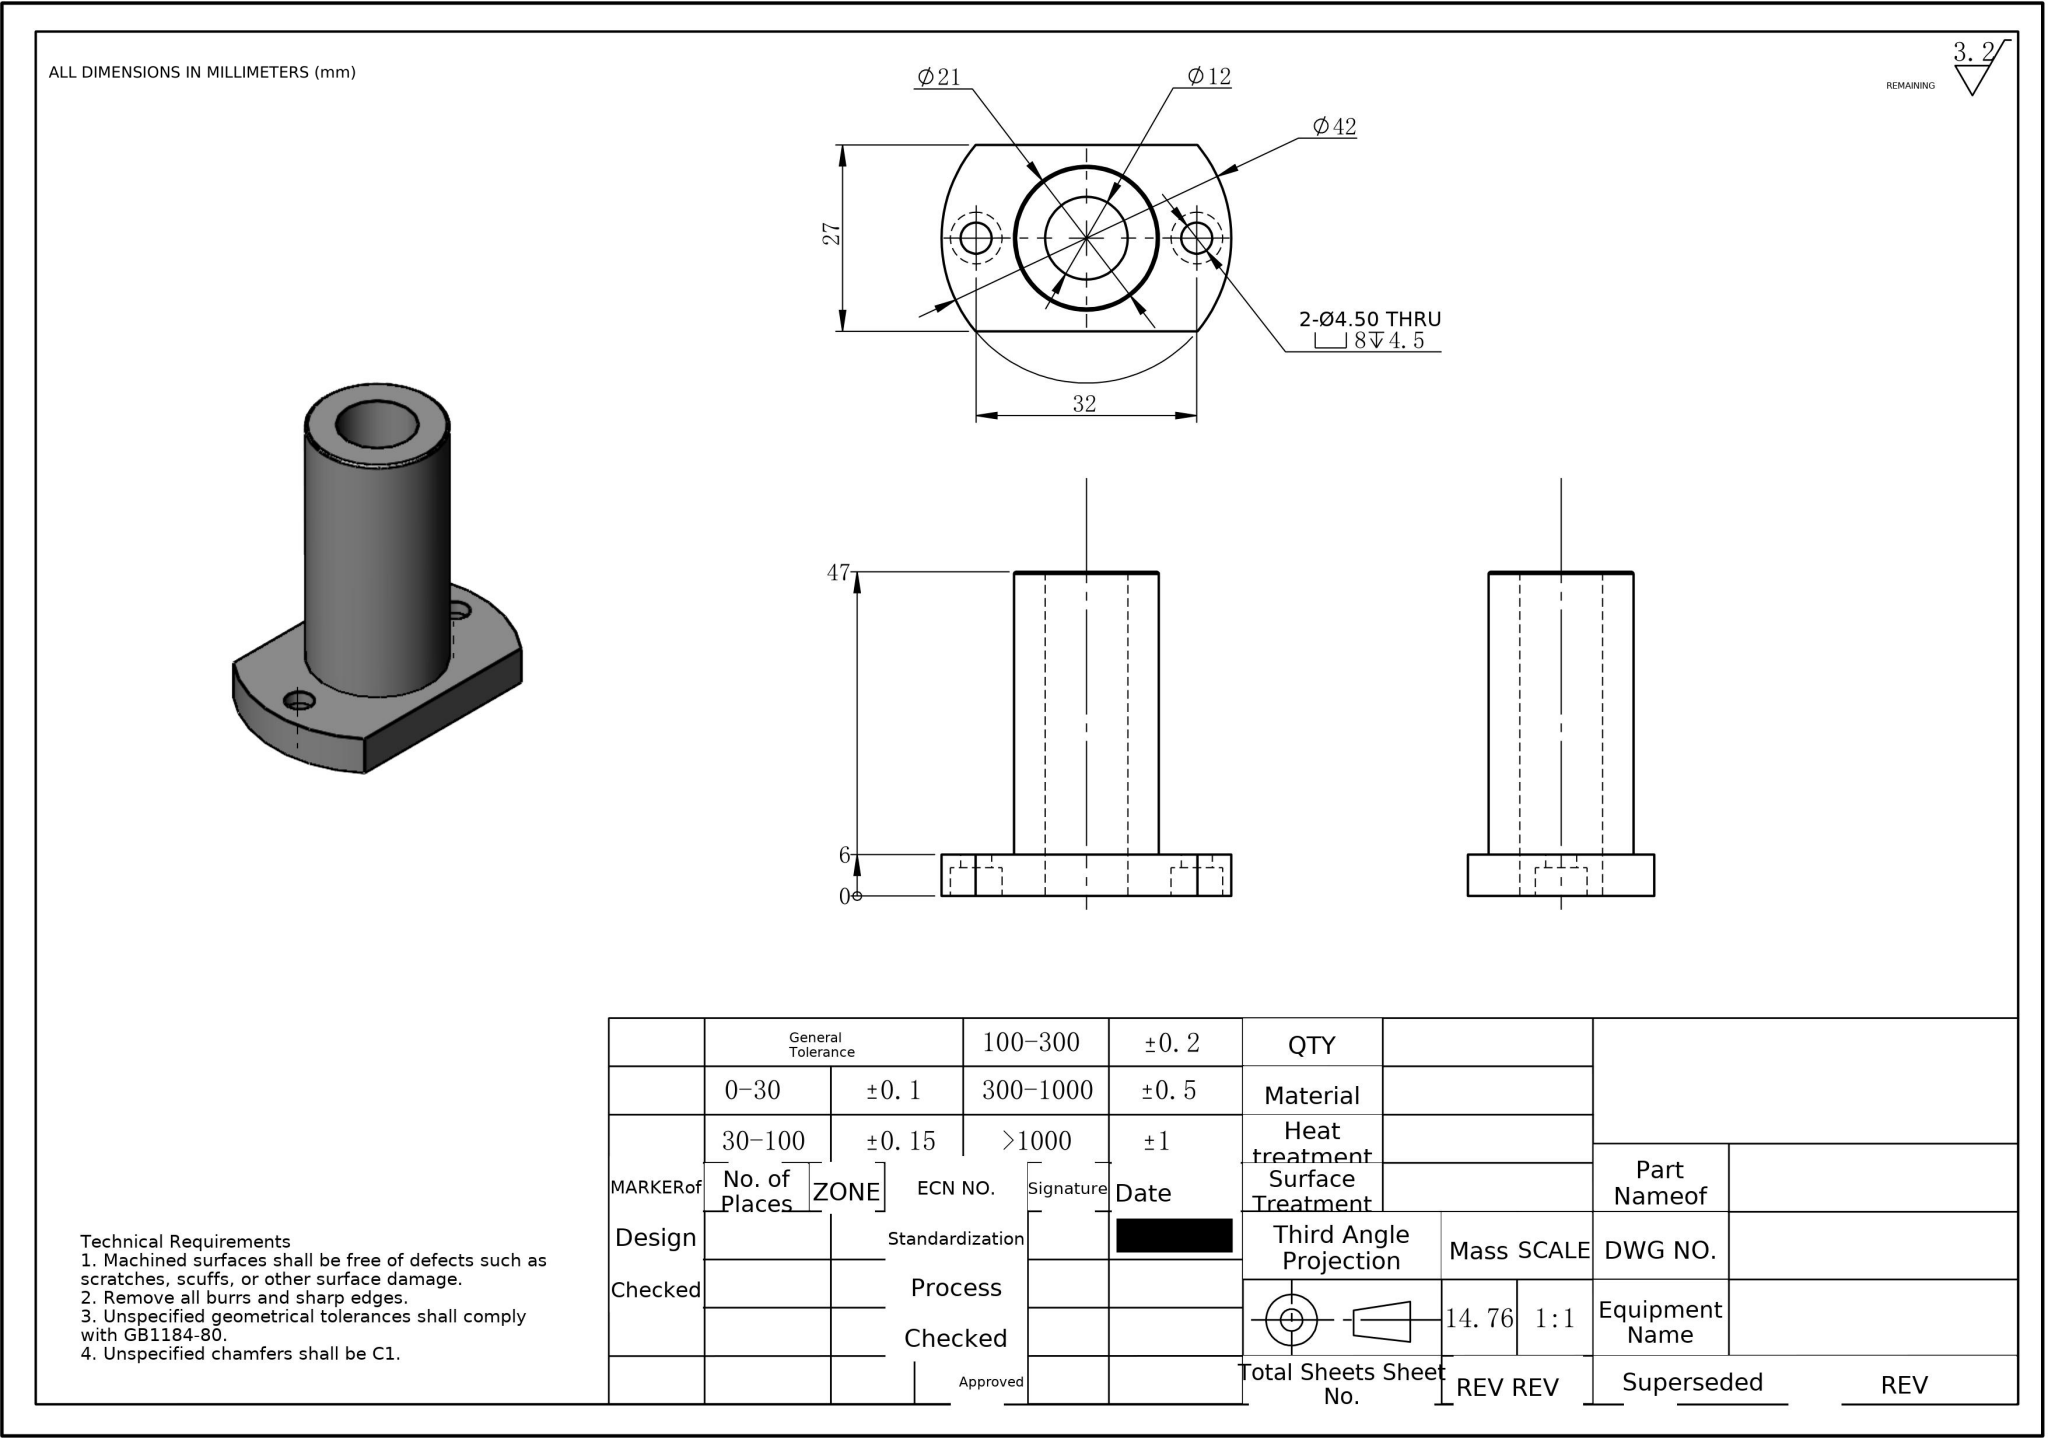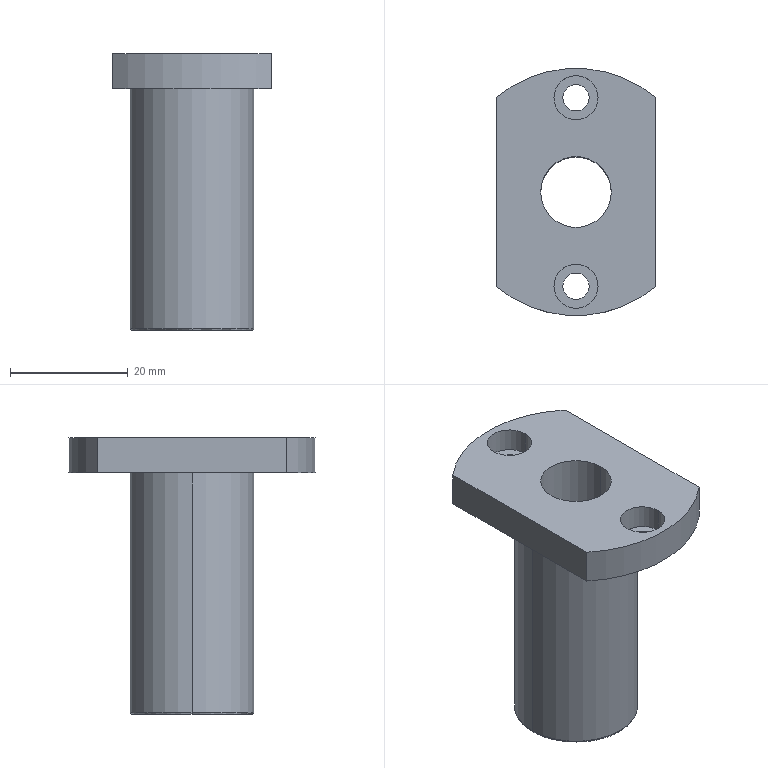Part | NX | mm | 1 solid | 23 faces | box 27 x 42 x 47 mm | volume 14763 mm3 | cylinder 14 | plane 7 | spline 2 | commonest cylinder face diameters 4.5 x4 7.5 x4 21 x2 12 x2 42 x2
STEP:
#1=COLOUR_RGB('',0.7922,0.8196,0.9333);
#2=FILL_AREA_STYLE_COLOUR('',#1);
#3=FILL_AREA_STYLE('',(#2));
#4=SURFACE_STYLE_FILL_AREA(#3);
#5=SURFACE_SIDE_STYLE('',(#4));
#6=SURFACE_STYLE_USAGE(.BOTH.,#5);
#7=PRESENTATION_STYLE_ASSIGNMENT((#6));
#8=CARTESIAN_POINT('',(-10.2,0.,-47.));
#9=VERTEX_POINT('',#8);
#10=CARTESIAN_POINT('',(10.2,0.,-47.));
#11=VERTEX_POINT('',#10);
#12=CARTESIAN_POINT('',(-10.2,0.,-47.));
#13=CARTESIAN_POINT('',(-10.2,-20.4,-47.));
#14=CARTESIAN_POINT('',(10.2,-20.4,-47.));
#15=CARTESIAN_POINT('',(10.2,0.,-47.));
#16=(BOUNDED_CURVE()B_SPLINE_CURVE(3,(#12,#13,#14,#15),.UNSPECIFIED.,.F.,.F.)B_SPLINE_CURVE_WITH_KNOTS((4,4),(0.,0.5),.UNSPECIFIED.)CURVE()GEOMETRIC_REPRESENTATION_ITEM()RATIONAL_B_SPLINE_CURVE((1.,0.3333,0.3333,1.))REPRESENTATION_ITEM(''));
#17=EDGE_CURVE('',#9,#11,#16,.T.);
#18=ORIENTED_EDGE('',*,*,#17,.T.);
#19=CARTESIAN_POINT('',(10.5,0.,-46.7));
#20=VERTEX_POINT('',#19);
#21=CARTESIAN_POINT('',(10.2,0.,-46.7));
#22=DIRECTION('',(0.,-1.,0.));
#23=DIRECTION('',(1.,0.,0.));
#24=AXIS2_PLACEMENT_3D('',#21,#22,#23);
#25=CIRCLE('',#24,0.3);
#26=EDGE_CURVE('',#11,#20,#25,.T.);
#27=ORIENTED_EDGE('',*,*,#26,.T.);
#28=CARTESIAN_POINT('',(-10.5,0.,-46.7));
#29=VERTEX_POINT('',#28);
#30=CARTESIAN_POINT('',(0.,0.,-46.7));
#31=DIRECTION('',(0.,0.,1.));
#32=DIRECTION('',(1.,0.,0.));
#33=AXIS2_PLACEMENT_3D('',#30,#31,#32);
#34=CIRCLE('',#33,10.5);
#35=EDGE_CURVE('',#29,#20,#34,.T.);
#36=ORIENTED_EDGE('',*,*,#35,.F.);
#37=CARTESIAN_POINT('',(-10.2,0.,-46.7));
#38=DIRECTION('',(0.,1.,0.));
#39=DIRECTION('',(-1.,0.,0.));
#40=AXIS2_PLACEMENT_3D('',#37,#38,#39);
#41=CIRCLE('',#40,0.3);
#42=EDGE_CURVE('',#9,#29,#41,.T.);
#43=ORIENTED_EDGE('',*,*,#42,.F.);
#44=EDGE_LOOP('',(#18,#27,#36,#43));
#45=FACE_OUTER_BOUND('',#44,.T.);
#46=CARTESIAN_POINT('',(10.2,0.,-47.));
#47=CARTESIAN_POINT('',(10.2,-20.4,-47.));
#48=CARTESIAN_POINT('',(-10.2,-20.4,-47.));
#49=CARTESIAN_POINT('',(-10.2,-0.,-47.));
#50=CARTESIAN_POINT('',(10.376,0.,-47.));
#51=CARTESIAN_POINT('',(10.376,-20.751,-47.));
#52=CARTESIAN_POINT('',(-10.376,-20.751,-47.));
#53=CARTESIAN_POINT('',(-10.376,-0.,-47.));
#54=CARTESIAN_POINT('',(10.5,0.,-46.876));
#55=CARTESIAN_POINT('',(10.5,-21.,-46.876));
#56=CARTESIAN_POINT('',(-10.5,-21.,-46.876));
#57=CARTESIAN_POINT('',(-10.5,-0.,-46.876));
#58=CARTESIAN_POINT('',(10.5,0.,-46.7));
#59=CARTESIAN_POINT('',(10.5,-21.,-46.7));
#60=CARTESIAN_POINT('',(-10.5,-21.,-46.7));
#61=CARTESIAN_POINT('',(-10.5,-0.,-46.7));
#62=(BOUNDED_SURFACE()B_SPLINE_SURFACE(3,3,((#46,#47,#48,#49),(#50,#51,#52,#53),(#54,#55,#56,#57),(#58,#59,#60,#61)),.UNSPECIFIED.,.F.,.F.,.T.)B_SPLINE_SURFACE_WITH_KNOTS((4,4),(4,4),(0.,1.),(0.,1.),.UNSPECIFIED.)GEOMETRIC_REPRESENTATION_ITEM()RATIONAL_B_SPLINE_SURFACE(((1.,0.3333,0.3333,1.),(0.8047,0.2682,0.2682,0.8047),(0.8047,0.2682,0.2682,0.8047),(1.,0.3333,0.3333,1.)))REPRESENTATION_ITEM('')SURFACE());
#63=ADVANCED_FACE('',(#45),#62,.T.);
#64=CARTESIAN_POINT('',(0.,0.,-46.7));
#65=DIRECTION('',(0.,0.,1.));
#66=DIRECTION('',(1.,0.,0.));
#67=AXIS2_PLACEMENT_3D('',#64,#65,#66);
#68=CIRCLE('',#67,10.5);
#69=EDGE_CURVE('',#20,#29,#68,.T.);
#70=ORIENTED_EDGE('',*,*,#69,.T.);
#71=CARTESIAN_POINT('',(-10.5,0.,-6.));
#72=VERTEX_POINT('',#71);
#73=CARTESIAN_POINT('',(-10.5,0.,-50.));
#74=DIRECTION('',(0.,0.,1.));
#75=VECTOR('',#74,1000.);
#76=LINE('',#73,#75);
#77=EDGE_CURVE('',#29,#72,#76,.T.);
#78=ORIENTED_EDGE('',*,*,#77,.T.);
#79=CARTESIAN_POINT('',(10.5,0.,-6.));
#80=VERTEX_POINT('',#79);
#81=CARTESIAN_POINT('',(0.,0.,-6.));
#82=DIRECTION('',(0.,0.,-1.));
#83=DIRECTION('',(1.,0.,0.));
#84=AXIS2_PLACEMENT_3D('',#81,#82,#83);
#85=CIRCLE('',#84,10.5);
#86=EDGE_CURVE('',#72,#80,#85,.T.);
#87=ORIENTED_EDGE('',*,*,#86,.T.);
#88=CARTESIAN_POINT('',(10.5,0.,-50.));
#89=DIRECTION('',(0.,0.,1.));
#90=VECTOR('',#89,1000.);
#91=LINE('',#88,#90);
#92=EDGE_CURVE('',#20,#80,#91,.T.);
#93=ORIENTED_EDGE('',*,*,#92,.F.);
#94=EDGE_LOOP('',(#70,#78,#87,#93));
#95=FACE_OUTER_BOUND('',#94,.T.);
#96=CARTESIAN_POINT('',(0.,0.,-50.));
#97=DIRECTION('',(0.,0.,1.));
#98=DIRECTION('',(1.,0.,0.));
#99=AXIS2_PLACEMENT_3D('',#96,#97,#98);
#100=CYLINDRICAL_SURFACE('',#99,10.5);
#101=ADVANCED_FACE('',(#95),#100,.T.);
#102=CARTESIAN_POINT('',(2.25,-16.,-6.));
#103=VERTEX_POINT('',#102);
#104=CARTESIAN_POINT('',(-2.25,-16.,-6.));
#105=VERTEX_POINT('',#104);
#106=CARTESIAN_POINT('',(0.,-16.,-6.));
#107=DIRECTION('',(0.,0.,-1.));
#108=DIRECTION('',(1.,0.,0.));
#109=AXIS2_PLACEMENT_3D('',#106,#107,#108);
#110=CIRCLE('',#109,2.25);
#111=EDGE_CURVE('',#103,#105,#110,.T.);
#112=ORIENTED_EDGE('',*,*,#111,.T.);
#113=CARTESIAN_POINT('',(-2.25,-16.,-4.1));
#114=VERTEX_POINT('',#113);
#115=CARTESIAN_POINT('',(-2.25,-16.,-6.));
#116=DIRECTION('',(0.,0.,1.));
#117=VECTOR('',#116,1000.);
#118=LINE('',#115,#117);
#119=EDGE_CURVE('',#105,#114,#118,.T.);
#120=ORIENTED_EDGE('',*,*,#119,.T.);
#121=CARTESIAN_POINT('',(2.25,-16.,-4.1));
#122=VERTEX_POINT('',#121);
#123=CARTESIAN_POINT('',(0.,-16.,-4.1));
#124=DIRECTION('',(0.,0.,-1.));
#125=DIRECTION('',(1.,0.,0.));
#126=AXIS2_PLACEMENT_3D('',#123,#124,#125);
#127=CIRCLE('',#126,2.25);
#128=EDGE_CURVE('',#122,#114,#127,.T.);
#129=ORIENTED_EDGE('',*,*,#128,.F.);
#130=CARTESIAN_POINT('',(2.25,-16.,-6.));
#131=DIRECTION('',(0.,0.,1.));
#132=VECTOR('',#131,1000.);
#133=LINE('',#130,#132);
#134=EDGE_CURVE('',#103,#122,#133,.T.);
#135=ORIENTED_EDGE('',*,*,#134,.F.);
#136=EDGE_LOOP('',(#112,#120,#129,#135));
#137=FACE_OUTER_BOUND('',#136,.T.);
#138=CARTESIAN_POINT('',(0.,-16.,-6.));
#139=DIRECTION('',(0.,0.,1.));
#140=DIRECTION('',(1.,0.,0.));
#141=AXIS2_PLACEMENT_3D('',#138,#139,#140);
#142=CYLINDRICAL_SURFACE('',#141,2.25);
#143=ADVANCED_FACE('',(#137),#142,.F.);
#144=CARTESIAN_POINT('',(2.25,16.,-6.));
#145=VERTEX_POINT('',#144);
#146=CARTESIAN_POINT('',(-2.25,16.,-6.));
#147=VERTEX_POINT('',#146);
#148=CARTESIAN_POINT('',(0.,16.,-6.));
#149=DIRECTION('',(0.,0.,-1.));
#150=DIRECTION('',(1.,0.,0.));
#151=AXIS2_PLACEMENT_3D('',#148,#149,#150);
#152=CIRCLE('',#151,2.25);
#153=EDGE_CURVE('',#145,#147,#152,.T.);
#154=ORIENTED_EDGE('',*,*,#153,.T.);
#155=CARTESIAN_POINT('',(-2.25,16.,-4.1));
#156=VERTEX_POINT('',#155);
#157=CARTESIAN_POINT('',(-2.25,16.,-6.));
#158=DIRECTION('',(0.,0.,1.));
#159=VECTOR('',#158,1000.);
#160=LINE('',#157,#159);
#161=EDGE_CURVE('',#147,#156,#160,.T.);
#162=ORIENTED_EDGE('',*,*,#161,.T.);
#163=CARTESIAN_POINT('',(2.25,16.,-4.1));
#164=VERTEX_POINT('',#163);
#165=CARTESIAN_POINT('',(0.,16.,-4.1));
#166=DIRECTION('',(0.,0.,-1.));
#167=DIRECTION('',(1.,0.,0.));
#168=AXIS2_PLACEMENT_3D('',#165,#166,#167);
#169=CIRCLE('',#168,2.25);
#170=EDGE_CURVE('',#164,#156,#169,.T.);
#171=ORIENTED_EDGE('',*,*,#170,.F.);
#172=CARTESIAN_POINT('',(2.25,16.,-6.));
#173=DIRECTION('',(0.,0.,1.));
#174=VECTOR('',#173,1000.);
#175=LINE('',#172,#174);
#176=EDGE_CURVE('',#145,#164,#175,.T.);
#177=ORIENTED_EDGE('',*,*,#176,.F.);
#178=EDGE_LOOP('',(#154,#162,#171,#177));
#179=FACE_OUTER_BOUND('',#178,.T.);
#180=CARTESIAN_POINT('',(0.,16.,-6.));
#181=DIRECTION('',(0.,0.,1.));
#182=DIRECTION('',(1.,0.,0.));
#183=AXIS2_PLACEMENT_3D('',#180,#181,#182);
#184=CYLINDRICAL_SURFACE('',#183,2.25);
#185=ADVANCED_FACE('',(#179),#184,.F.);
#186=CARTESIAN_POINT('',(-6.,0.,-47.));
#187=VERTEX_POINT('',#186);
#188=CARTESIAN_POINT('',(6.,0.,-47.));
#189=VERTEX_POINT('',#188);
#190=CARTESIAN_POINT('',(0.,0.,-47.));
#191=DIRECTION('',(0.,0.,1.));
#192=DIRECTION('',(1.,0.,0.));
#193=AXIS2_PLACEMENT_3D('',#190,#191,#192);
#194=CIRCLE('',#193,6.);
#195=EDGE_CURVE('',#187,#189,#194,.T.);
#196=ORIENTED_EDGE('',*,*,#195,.F.);
#197=CARTESIAN_POINT('',(-6.,0.,0.));
#198=VERTEX_POINT('',#197);
#199=CARTESIAN_POINT('',(-6.,0.,-50.));
#200=DIRECTION('',(0.,0.,1.));
#201=VECTOR('',#200,1000.);
#202=LINE('',#199,#201);
#203=EDGE_CURVE('',#187,#198,#202,.T.);
#204=ORIENTED_EDGE('',*,*,#203,.T.);
#205=CARTESIAN_POINT('',(6.,0.,0.));
#206=VERTEX_POINT('',#205);
#207=CARTESIAN_POINT('',(0.,0.,0.));
#208=DIRECTION('',(0.,0.,-1.));
#209=DIRECTION('',(1.,0.,0.));
#210=AXIS2_PLACEMENT_3D('',#207,#208,#209);
#211=CIRCLE('',#210,6.);
#212=EDGE_CURVE('',#206,#198,#211,.T.);
#213=ORIENTED_EDGE('',*,*,#212,.F.);
#214=CARTESIAN_POINT('',(6.,0.,-50.));
#215=DIRECTION('',(0.,0.,1.));
#216=VECTOR('',#215,1000.);
#217=LINE('',#214,#216);
#218=EDGE_CURVE('',#189,#206,#217,.T.);
#219=ORIENTED_EDGE('',*,*,#218,.F.);
#220=EDGE_LOOP('',(#196,#204,#213,#219));
#221=FACE_OUTER_BOUND('',#220,.T.);
#222=CARTESIAN_POINT('',(0.,0.,-50.));
#223=DIRECTION('',(0.,0.,1.));
#224=DIRECTION('',(1.,0.,0.));
#225=AXIS2_PLACEMENT_3D('',#222,#223,#224);
#226=CYLINDRICAL_SURFACE('',#225,6.);
#227=ADVANCED_FACE('',(#221),#226,.F.);
#228=CARTESIAN_POINT('',(-3.75,-16.,-4.1));
#229=VERTEX_POINT('',#228);
#230=CARTESIAN_POINT('',(3.75,-16.,-4.1));
#231=VERTEX_POINT('',#230);
#232=CARTESIAN_POINT('',(0.,-16.,-4.1));
#233=DIRECTION('',(0.,0.,1.));
#234=DIRECTION('',(1.,0.,0.));
#235=AXIS2_PLACEMENT_3D('',#232,#233,#234);
#236=CIRCLE('',#235,3.75);
#237=EDGE_CURVE('',#229,#231,#236,.T.);
#238=ORIENTED_EDGE('',*,*,#237,.F.);
#239=CARTESIAN_POINT('',(-3.75,-16.,0.));
#240=VERTEX_POINT('',#239);
#241=CARTESIAN_POINT('',(-3.75,-16.,-6.));
#242=DIRECTION('',(0.,0.,1.));
#243=VECTOR('',#242,1000.);
#244=LINE('',#241,#243);
#245=EDGE_CURVE('',#229,#240,#244,.T.);
#246=ORIENTED_EDGE('',*,*,#245,.T.);
#247=CARTESIAN_POINT('',(3.75,-16.,0.));
#248=VERTEX_POINT('',#247);
#249=CARTESIAN_POINT('',(0.,-16.,0.));
#250=DIRECTION('',(0.,0.,-1.));
#251=DIRECTION('',(1.,0.,0.));
#252=AXIS2_PLACEMENT_3D('',#249,#250,#251);
#253=CIRCLE('',#252,3.75);
#254=EDGE_CURVE('',#248,#240,#253,.T.);
#255=ORIENTED_EDGE('',*,*,#254,.F.);
#256=CARTESIAN_POINT('',(3.75,-16.,-6.));
#257=DIRECTION('',(0.,0.,1.));
#258=VECTOR('',#257,1000.);
#259=LINE('',#256,#258);
#260=EDGE_CURVE('',#231,#248,#259,.T.);
#261=ORIENTED_EDGE('',*,*,#260,.F.);
#262=EDGE_LOOP('',(#238,#246,#255,#261));
#263=FACE_OUTER_BOUND('',#262,.T.);
#264=CARTESIAN_POINT('',(0.,-16.,-6.));
#265=DIRECTION('',(0.,0.,1.));
#266=DIRECTION('',(1.,0.,0.));
#267=AXIS2_PLACEMENT_3D('',#264,#265,#266);
#268=CYLINDRICAL_SURFACE('',#267,3.75);
#269=ADVANCED_FACE('',(#263),#268,.F.);
#270=CARTESIAN_POINT('',(-3.75,16.,-4.1));
#271=VERTEX_POINT('',#270);
#272=CARTESIAN_POINT('',(3.75,16.,-4.1));
#273=VERTEX_POINT('',#272);
#274=CARTESIAN_POINT('',(0.,16.,-4.1));
#275=DIRECTION('',(0.,0.,1.));
#276=DIRECTION('',(1.,0.,0.));
#277=AXIS2_PLACEMENT_3D('',#274,#275,#276);
#278=CIRCLE('',#277,3.75);
#279=EDGE_CURVE('',#271,#273,#278,.T.);
#280=ORIENTED_EDGE('',*,*,#279,.F.);
#281=CARTESIAN_POINT('',(-3.75,16.,0.));
#282=VERTEX_POINT('',#281);
#283=CARTESIAN_POINT('',(-3.75,16.,-6.));
#284=DIRECTION('',(0.,0.,1.));
#285=VECTOR('',#284,1000.);
#286=LINE('',#283,#285);
#287=EDGE_CURVE('',#271,#282,#286,.T.);
#288=ORIENTED_EDGE('',*,*,#287,.T.);
#289=CARTESIAN_POINT('',(3.75,16.,0.));
#290=VERTEX_POINT('',#289);
#291=CARTESIAN_POINT('',(0.,16.,0.));
#292=DIRECTION('',(0.,0.,-1.));
#293=DIRECTION('',(1.,0.,0.));
#294=AXIS2_PLACEMENT_3D('',#291,#292,#293);
#295=CIRCLE('',#294,3.75);
#296=EDGE_CURVE('',#290,#282,#295,.T.);
#297=ORIENTED_EDGE('',*,*,#296,.F.);
#298=CARTESIAN_POINT('',(3.75,16.,-6.));
#299=DIRECTION('',(0.,0.,1.));
#300=VECTOR('',#299,1000.);
#301=LINE('',#298,#300);
#302=EDGE_CURVE('',#273,#290,#301,.T.);
#303=ORIENTED_EDGE('',*,*,#302,.F.);
#304=EDGE_LOOP('',(#280,#288,#297,#303));
#305=FACE_OUTER_BOUND('',#304,.T.);
#306=CARTESIAN_POINT('',(0.,16.,-6.));
#307=DIRECTION('',(0.,0.,1.));
#308=DIRECTION('',(1.,0.,0.));
#309=AXIS2_PLACEMENT_3D('',#306,#307,#308);
#310=CYLINDRICAL_SURFACE('',#309,3.75);
#311=ADVANCED_FACE('',(#305),#310,.F.);
#312=ORIENTED_EDGE('',*,*,#77,.F.);
#313=ORIENTED_EDGE('',*,*,#35,.T.);
#314=ORIENTED_EDGE('',*,*,#92,.T.);
#315=CARTESIAN_POINT('',(0.,0.,-6.));
#316=DIRECTION('',(0.,0.,-1.));
#317=DIRECTION('',(1.,0.,0.));
#318=AXIS2_PLACEMENT_3D('',#315,#316,#317);
#319=CIRCLE('',#318,10.5);
#320=EDGE_CURVE('',#80,#72,#319,.T.);
#321=ORIENTED_EDGE('',*,*,#320,.T.);
#322=EDGE_LOOP('',(#312,#313,#314,#321));
#323=FACE_OUTER_BOUND('',#322,.T.);
#324=CARTESIAN_POINT('',(0.,0.,-50.));
#325=DIRECTION('',(0.,0.,1.));
#326=DIRECTION('',(1.,0.,0.));
#327=AXIS2_PLACEMENT_3D('',#324,#325,#326);
#328=CYLINDRICAL_SURFACE('',#327,10.5);
#329=ADVANCED_FACE('',(#323),#328,.T.);
#330=ORIENTED_EDGE('',*,*,#26,.F.);
#331=CARTESIAN_POINT('',(10.2,0.,-47.));
#332=CARTESIAN_POINT('',(10.2,20.4,-47.));
#333=CARTESIAN_POINT('',(-10.2,20.4,-47.));
#334=CARTESIAN_POINT('',(-10.2,0.,-47.));
#335=(BOUNDED_CURVE()B_SPLINE_CURVE(3,(#331,#332,#333,#334),.UNSPECIFIED.,.F.,.F.)B_SPLINE_CURVE_WITH_KNOTS((4,4),(0.5,1.),.UNSPECIFIED.)CURVE()GEOMETRIC_REPRESENTATION_ITEM()RATIONAL_B_SPLINE_CURVE((1.,0.3333,0.3333,1.))REPRESENTATION_ITEM(''));
#336=EDGE_CURVE('',#11,#9,#335,.T.);
#337=ORIENTED_EDGE('',*,*,#336,.T.);
#338=ORIENTED_EDGE('',*,*,#42,.T.);
#339=ORIENTED_EDGE('',*,*,#69,.F.);
#340=EDGE_LOOP('',(#330,#337,#338,#339));
#341=FACE_OUTER_BOUND('',#340,.T.);
#342=CARTESIAN_POINT('',(-10.2,0.,-47.));
#343=CARTESIAN_POINT('',(-10.2,20.4,-47.));
#344=CARTESIAN_POINT('',(10.2,20.4,-47.));
#345=CARTESIAN_POINT('',(10.2,0.,-47.));
#346=CARTESIAN_POINT('',(-10.376,0.,-47.));
#347=CARTESIAN_POINT('',(-10.376,20.751,-47.));
#348=CARTESIAN_POINT('',(10.376,20.751,-47.));
#349=CARTESIAN_POINT('',(10.376,0.,-47.));
#350=CARTESIAN_POINT('',(-10.5,0.,-46.876));
#351=CARTESIAN_POINT('',(-10.5,21.,-46.876));
#352=CARTESIAN_POINT('',(10.5,21.,-46.876));
#353=CARTESIAN_POINT('',(10.5,0.,-46.876));
#354=CARTESIAN_POINT('',(-10.5,0.,-46.7));
#355=CARTESIAN_POINT('',(-10.5,21.,-46.7));
#356=CARTESIAN_POINT('',(10.5,21.,-46.7));
#357=CARTESIAN_POINT('',(10.5,0.,-46.7));
#358=(BOUNDED_SURFACE()B_SPLINE_SURFACE(3,3,((#342,#343,#344,#345),(#346,#347,#348,#349),(#350,#351,#352,#353),(#354,#355,#356,#357)),.UNSPECIFIED.,.F.,.F.,.T.)B_SPLINE_SURFACE_WITH_KNOTS((4,4),(4,4),(0.,1.),(0.,1.),.UNSPECIFIED.)GEOMETRIC_REPRESENTATION_ITEM()RATIONAL_B_SPLINE_SURFACE(((1.,0.3333,0.3333,1.),(0.8047,0.2682,0.2682,0.8047),(0.8047,0.2682,0.2682,0.8047),(1.,0.3333,0.3333,1.)))REPRESENTATION_ITEM('')SURFACE());
#359=ADVANCED_FACE('',(#341),#358,.T.);
#360=ORIENTED_EDGE('',*,*,#111,.F.);
#361=CARTESIAN_POINT('',(0.,-16.,-6.));
#362=DIRECTION('',(0.,0.,-1.));
#363=DIRECTION('',(1.,0.,0.));
#364=AXIS2_PLACEMENT_3D('',#361,#362,#363);
#365=CIRCLE('',#364,2.25);
#366=EDGE_CURVE('',#105,#103,#365,.T.);
#367=ORIENTED_EDGE('',*,*,#366,.F.);
#368=EDGE_LOOP('',(#360,#367));
#369=FACE_BOUND('',#368,.T.);
#370=CARTESIAN_POINT('',(13.5,16.086,-6.));
#371=VERTEX_POINT('',#370);
#372=CARTESIAN_POINT('',(-13.5,16.086,-6.));
#373=VERTEX_POINT('',#372);
#374=CARTESIAN_POINT('',(0.,0.,-6.));
#375=DIRECTION('',(0.,0.,1.));
#376=DIRECTION('',(-1.,0.,0.));
#377=AXIS2_PLACEMENT_3D('',#374,#375,#376);
#378=CIRCLE('',#377,21.);
#379=EDGE_CURVE('',#371,#373,#378,.T.);
#380=ORIENTED_EDGE('',*,*,#379,.F.);
#381=CARTESIAN_POINT('',(13.5,-16.086,-6.));
#382=VERTEX_POINT('',#381);
#383=CARTESIAN_POINT('',(13.5,-0.,-6.));
#384=DIRECTION('',(0.,1.,0.));
#385=VECTOR('',#384,1000.);
#386=LINE('',#383,#385);
#387=EDGE_CURVE('',#382,#371,#386,.T.);
#388=ORIENTED_EDGE('',*,*,#387,.F.);
#389=CARTESIAN_POINT('',(-13.5,-16.086,-6.));
#390=VERTEX_POINT('',#389);
#391=CARTESIAN_POINT('',(0.,-0.,-6.));
#392=DIRECTION('',(0.,0.,1.));
#393=DIRECTION('',(-1.,0.,0.));
#394=AXIS2_PLACEMENT_3D('',#391,#392,#393);
#395=CIRCLE('',#394,21.);
#396=EDGE_CURVE('',#390,#382,#395,.T.);
#397=ORIENTED_EDGE('',*,*,#396,.F.);
#398=CARTESIAN_POINT('',(-13.5,-0.,-6.));
#399=DIRECTION('',(0.,-1.,0.));
#400=VECTOR('',#399,1000.);
#401=LINE('',#398,#400);
#402=EDGE_CURVE('',#373,#390,#401,.T.);
#403=ORIENTED_EDGE('',*,*,#402,.F.);
#404=EDGE_LOOP('',(#380,#388,#397,#403));
#405=FACE_OUTER_BOUND('',#404,.T.);
#406=ORIENTED_EDGE('',*,*,#320,.F.);
#407=ORIENTED_EDGE('',*,*,#86,.F.);
#408=EDGE_LOOP('',(#406,#407));
#409=FACE_BOUND('',#408,.T.);
#410=ORIENTED_EDGE('',*,*,#153,.F.);
#411=CARTESIAN_POINT('',(0.,16.,-6.));
#412=DIRECTION('',(0.,0.,-1.));
#413=DIRECTION('',(1.,0.,0.));
#414=AXIS2_PLACEMENT_3D('',#411,#412,#413);
#415=CIRCLE('',#414,2.25);
#416=EDGE_CURVE('',#147,#145,#415,.T.);
#417=ORIENTED_EDGE('',*,*,#416,.F.);
#418=EDGE_LOOP('',(#410,#417));
#419=FACE_BOUND('',#418,.T.);
#420=CARTESIAN_POINT('',(0.,-0.,-6.));
#421=DIRECTION('',(0.,0.,1.));
#422=DIRECTION('',(1.,0.,0.));
#423=AXIS2_PLACEMENT_3D('',#420,#421,#422);
#424=PLANE('',#423);
#425=ADVANCED_FACE('',(#369,#405,#409,#419),#424,.F.);
#426=CARTESIAN_POINT('',(0.,0.,-47.));
#427=DIRECTION('',(0.,0.,1.));
#428=DIRECTION('',(1.,0.,0.));
#429=AXIS2_PLACEMENT_3D('',#426,#427,#428);
#430=CIRCLE('',#429,6.);
#431=EDGE_CURVE('',#189,#187,#430,.T.);
#432=ORIENTED_EDGE('',*,*,#431,.T.);
#433=ORIENTED_EDGE('',*,*,#195,.T.);
#434=EDGE_LOOP('',(#432,#433));
#435=FACE_BOUND('',#434,.T.);
#436=ORIENTED_EDGE('',*,*,#17,.F.);
#437=ORIENTED_EDGE('',*,*,#336,.F.);
#438=EDGE_LOOP('',(#436,#437));
#439=FACE_OUTER_BOUND('',#438,.T.);
#440=CARTESIAN_POINT('',(0.,6.,-47.));
#441=DIRECTION('',(0.,0.,-1.));
#442=DIRECTION('',(-1.,0.,0.));
#443=AXIS2_PLACEMENT_3D('',#440,#441,#442);
#444=PLANE('',#443);
#445=ADVANCED_FACE('',(#435,#439),#444,.T.);
#446=ORIENTED_EDGE('',*,*,#119,.F.);
#447=ORIENTED_EDGE('',*,*,#366,.T.);
#448=ORIENTED_EDGE('',*,*,#134,.T.);
#449=CARTESIAN_POINT('',(0.,-16.,-4.1));
#450=DIRECTION('',(0.,0.,-1.));
#451=DIRECTION('',(1.,0.,0.));
#452=AXIS2_PLACEMENT_3D('',#449,#450,#451);
#453=CIRCLE('',#452,2.25);
#454=EDGE_CURVE('',#114,#122,#453,.T.);
#455=ORIENTED_EDGE('',*,*,#454,.F.);
#456=EDGE_LOOP('',(#446,#447,#448,#455));
#457=FACE_OUTER_BOUND('',#456,.T.);
#458=CARTESIAN_POINT('',(0.,-16.,-6.));
#459=DIRECTION('',(0.,0.,1.));
#460=DIRECTION('',(1.,0.,0.));
#461=AXIS2_PLACEMENT_3D('',#458,#459,#460);
#462=CYLINDRICAL_SURFACE('',#461,2.25);
#463=ADVANCED_FACE('',(#457),#462,.F.);
#464=ORIENTED_EDGE('',*,*,#402,.T.);
#465=CARTESIAN_POINT('',(-13.5,-16.086,0.));
#466=VERTEX_POINT('',#465);
#467=CARTESIAN_POINT('',(-13.5,-16.086,-6.));
#468=DIRECTION('',(0.,0.,1.));
#469=VECTOR('',#468,1000.);
#470=LINE('',#467,#469);
#471=EDGE_CURVE('',#390,#466,#470,.T.);
#472=ORIENTED_EDGE('',*,*,#471,.T.);
#473=CARTESIAN_POINT('',(-13.5,16.086,0.));
#474=VERTEX_POINT('',#473);
#475=CARTESIAN_POINT('',(-13.5,16.086,0.));
#476=DIRECTION('',(0.,1.,0.));
#477=VECTOR('',#476,1000.);
#478=LINE('',#475,#477);
#479=EDGE_CURVE('',#466,#474,#478,.T.);
#480=ORIENTED_EDGE('',*,*,#479,.T.);
#481=CARTESIAN_POINT('',(-13.5,16.086,-6.));
#482=DIRECTION('',(0.,0.,-1.));
#483=VECTOR('',#482,1000.);
#484=LINE('',#481,#483);
#485=EDGE_CURVE('',#474,#373,#484,.T.);
#486=ORIENTED_EDGE('',*,*,#485,.T.);
#487=EDGE_LOOP('',(#464,#472,#480,#486));
#488=FACE_OUTER_BOUND('',#487,.T.);
#489=CARTESIAN_POINT('',(-13.5,16.086,-6.));
#490=DIRECTION('',(-1.,0.,0.));
#491=DIRECTION('',(0.,0.,1.));
#492=AXIS2_PLACEMENT_3D('',#489,#490,#491);
#493=PLANE('',#492);
#494=ADVANCED_FACE('',(#488),#493,.T.);
#495=ORIENTED_EDGE('',*,*,#379,.T.);
#496=ORIENTED_EDGE('',*,*,#485,.F.);
#497=CARTESIAN_POINT('',(13.5,16.086,0.));
#498=VERTEX_POINT('',#497);
#499=CARTESIAN_POINT('',(0.,0.,0.));
#500=DIRECTION('',(0.,0.,-1.));
#501=DIRECTION('',(-1.,0.,0.));
#502=AXIS2_PLACEMENT_3D('',#499,#500,#501);
#503=CIRCLE('',#502,21.);
#504=EDGE_CURVE('',#474,#498,#503,.T.);
#505=ORIENTED_EDGE('',*,*,#504,.T.);
#506=CARTESIAN_POINT('',(13.5,16.086,-6.));
#507=DIRECTION('',(0.,0.,-1.));
#508=VECTOR('',#507,1000.);
#509=LINE('',#506,#508);
#510=EDGE_CURVE('',#498,#371,#509,.T.);
#511=ORIENTED_EDGE('',*,*,#510,.T.);
#512=EDGE_LOOP('',(#495,#496,#505,#511));
#513=FACE_OUTER_BOUND('',#512,.T.);
#514=CARTESIAN_POINT('',(0.,0.,-6.));
#515=DIRECTION('',(0.,0.,-1.));
#516=DIRECTION('',(-1.,0.,0.));
#517=AXIS2_PLACEMENT_3D('',#514,#515,#516);
#518=CYLINDRICAL_SURFACE('',#517,21.);
#519=ADVANCED_FACE('',(#513),#518,.T.);
#520=ORIENTED_EDGE('',*,*,#387,.T.);
#521=ORIENTED_EDGE('',*,*,#510,.F.);
#522=CARTESIAN_POINT('',(13.5,-16.086,0.));
#523=VERTEX_POINT('',#522);
#524=CARTESIAN_POINT('',(13.5,-16.086,0.));
#525=DIRECTION('',(0.,-1.,0.));
#526=VECTOR('',#525,1000.);
#527=LINE('',#524,#526);
#528=EDGE_CURVE('',#498,#523,#527,.T.);
#529=ORIENTED_EDGE('',*,*,#528,.T.);
#530=CARTESIAN_POINT('',(13.5,-16.086,-6.));
#531=DIRECTION('',(0.,0.,-1.));
#532=VECTOR('',#531,1000.);
#533=LINE('',#530,#532);
#534=EDGE_CURVE('',#523,#382,#533,.T.);
#535=ORIENTED_EDGE('',*,*,#534,.T.);
#536=EDGE_LOOP('',(#520,#521,#529,#535));
#537=FACE_OUTER_BOUND('',#536,.T.);
#538=CARTESIAN_POINT('',(13.5,-16.086,-6.));
#539=DIRECTION('',(1.,0.,0.));
#540=DIRECTION('',(0.,0.,-1.));
#541=AXIS2_PLACEMENT_3D('',#538,#539,#540);
#542=PLANE('',#541);
#543=ADVANCED_FACE('',(#537),#542,.T.);
#544=ORIENTED_EDGE('',*,*,#396,.T.);
#545=ORIENTED_EDGE('',*,*,#534,.F.);
#546=CARTESIAN_POINT('',(0.,-0.,0.));
#547=DIRECTION('',(0.,0.,-1.));
#548=DIRECTION('',(-1.,0.,0.));
#549=AXIS2_PLACEMENT_3D('',#546,#547,#548);
#550=CIRCLE('',#549,21.);
#551=EDGE_CURVE('',#523,#466,#550,.T.);
#552=ORIENTED_EDGE('',*,*,#551,.T.);
#553=ORIENTED_EDGE('',*,*,#471,.F.);
#554=EDGE_LOOP('',(#544,#545,#552,#553));
#555=FACE_OUTER_BOUND('',#554,.T.);
#556=CARTESIAN_POINT('',(0.,-0.,-6.));
#557=DIRECTION('',(0.,0.,-1.));
#558=DIRECTION('',(-1.,0.,0.));
#559=AXIS2_PLACEMENT_3D('',#556,#557,#558);
#560=CYLINDRICAL_SURFACE('',#559,21.);
#561=ADVANCED_FACE('',(#555),#560,.T.);
#562=ORIENTED_EDGE('',*,*,#161,.F.);
#563=ORIENTED_EDGE('',*,*,#416,.T.);
#564=ORIENTED_EDGE('',*,*,#176,.T.);
#565=CARTESIAN_POINT('',(0.,16.,-4.1));
#566=DIRECTION('',(0.,0.,-1.));
#567=DIRECTION('',(1.,0.,0.));
#568=AXIS2_PLACEMENT_3D('',#565,#566,#567);
#569=CIRCLE('',#568,2.25);
#570=EDGE_CURVE('',#156,#164,#569,.T.);
#571=ORIENTED_EDGE('',*,*,#570,.F.);
#572=EDGE_LOOP('',(#562,#563,#564,#571));
#573=FACE_OUTER_BOUND('',#572,.T.);
#574=CARTESIAN_POINT('',(0.,16.,-6.));
#575=DIRECTION('',(0.,0.,1.));
#576=DIRECTION('',(1.,0.,0.));
#577=AXIS2_PLACEMENT_3D('',#574,#575,#576);
#578=CYLINDRICAL_SURFACE('',#577,2.25);
#579=ADVANCED_FACE('',(#573),#578,.F.);
#580=ORIENTED_EDGE('',*,*,#203,.F.);
#581=ORIENTED_EDGE('',*,*,#431,.F.);
#582=ORIENTED_EDGE('',*,*,#218,.T.);
#583=CARTESIAN_POINT('',(0.,0.,0.));
#584=DIRECTION('',(0.,0.,-1.));
#585=DIRECTION('',(1.,0.,0.));
#586=AXIS2_PLACEMENT_3D('',#583,#584,#585);
#587=CIRCLE('',#586,6.);
#588=EDGE_CURVE('',#198,#206,#587,.T.);
#589=ORIENTED_EDGE('',*,*,#588,.F.);
#590=EDGE_LOOP('',(#580,#581,#582,#589));
#591=FACE_OUTER_BOUND('',#590,.T.);
#592=CARTESIAN_POINT('',(0.,0.,-50.));
#593=DIRECTION('',(0.,0.,1.));
#594=DIRECTION('',(1.,0.,0.));
#595=AXIS2_PLACEMENT_3D('',#592,#593,#594);
#596=CYLINDRICAL_SURFACE('',#595,6.);
#597=ADVANCED_FACE('',(#591),#596,.F.);
#598=CARTESIAN_POINT('',(0.,-16.,-4.1));
#599=DIRECTION('',(0.,0.,1.));
#600=DIRECTION('',(1.,0.,0.));
#601=AXIS2_PLACEMENT_3D('',#598,#599,#600);
#602=CIRCLE('',#601,3.75);
#603=EDGE_CURVE('',#231,#229,#602,.T.);
#604=ORIENTED_EDGE('',*,*,#603,.T.);
#605=ORIENTED_EDGE('',*,*,#237,.T.);
#606=EDGE_LOOP('',(#604,#605));
#607=FACE_OUTER_BOUND('',#606,.T.);
#608=ORIENTED_EDGE('',*,*,#128,.T.);
#609=ORIENTED_EDGE('',*,*,#454,.T.);
#610=EDGE_LOOP('',(#608,#609));
#611=FACE_BOUND('',#610,.T.);
#612=CARTESIAN_POINT('',(0.,-12.25,-4.1));
#613=DIRECTION('',(0.,0.,1.));
#614=DIRECTION('',(1.,0.,0.));
#615=AXIS2_PLACEMENT_3D('',#612,#613,#614);
#616=PLANE('',#615);
#617=ADVANCED_FACE('',(#607,#611),#616,.T.);
#618=ORIENTED_EDGE('',*,*,#254,.T.);
#619=CARTESIAN_POINT('',(0.,-16.,0.));
#620=DIRECTION('',(0.,0.,-1.));
#621=DIRECTION('',(1.,0.,0.));
#622=AXIS2_PLACEMENT_3D('',#619,#620,#621);
#623=CIRCLE('',#622,3.75);
#624=EDGE_CURVE('',#240,#248,#623,.T.);
#625=ORIENTED_EDGE('',*,*,#624,.T.);
#626=EDGE_LOOP('',(#618,#625));
#627=FACE_BOUND('',#626,.T.);
#628=ORIENTED_EDGE('',*,*,#528,.F.);
#629=ORIENTED_EDGE('',*,*,#504,.F.);
#630=ORIENTED_EDGE('',*,*,#479,.F.);
#631=ORIENTED_EDGE('',*,*,#551,.F.);
#632=EDGE_LOOP('',(#628,#629,#630,#631));
#633=FACE_OUTER_BOUND('',#632,.T.);
#634=ORIENTED_EDGE('',*,*,#212,.T.);
#635=ORIENTED_EDGE('',*,*,#588,.T.);
#636=EDGE_LOOP('',(#634,#635));
#637=FACE_BOUND('',#636,.T.);
#638=ORIENTED_EDGE('',*,*,#296,.T.);
#639=CARTESIAN_POINT('',(0.,16.,0.));
#640=DIRECTION('',(0.,0.,-1.));
#641=DIRECTION('',(1.,0.,0.));
#642=AXIS2_PLACEMENT_3D('',#639,#640,#641);
#643=CIRCLE('',#642,3.75);
#644=EDGE_CURVE('',#282,#290,#643,.T.);
#645=ORIENTED_EDGE('',*,*,#644,.T.);
#646=EDGE_LOOP('',(#638,#645));
#647=FACE_BOUND('',#646,.T.);
#648=CARTESIAN_POINT('',(0.,-0.,0.));
#649=DIRECTION('',(0.,0.,1.));
#650=DIRECTION('',(1.,0.,0.));
#651=AXIS2_PLACEMENT_3D('',#648,#649,#650);
#652=PLANE('',#651);
#653=ADVANCED_FACE('',(#627,#633,#637,#647),#652,.T.);
#654=CARTESIAN_POINT('',(0.,16.,-4.1));
#655=DIRECTION('',(0.,0.,1.));
#656=DIRECTION('',(1.,0.,0.));
#657=AXIS2_PLACEMENT_3D('',#654,#655,#656);
#658=CIRCLE('',#657,3.75);
#659=EDGE_CURVE('',#273,#271,#658,.T.);
#660=ORIENTED_EDGE('',*,*,#659,.T.);
#661=ORIENTED_EDGE('',*,*,#279,.T.);
#662=EDGE_LOOP('',(#660,#661));
#663=FACE_OUTER_BOUND('',#662,.T.);
#664=ORIENTED_EDGE('',*,*,#170,.T.);
#665=ORIENTED_EDGE('',*,*,#570,.T.);
#666=EDGE_LOOP('',(#664,#665));
#667=FACE_BOUND('',#666,.T.);
#668=CARTESIAN_POINT('',(0.,19.75,-4.1));
#669=DIRECTION('',(0.,0.,1.));
#670=DIRECTION('',(1.,0.,0.));
#671=AXIS2_PLACEMENT_3D('',#668,#669,#670);
#672=PLANE('',#671);
#673=ADVANCED_FACE('',(#663,#667),#672,.T.);
#674=ORIENTED_EDGE('',*,*,#245,.F.);
#675=ORIENTED_EDGE('',*,*,#603,.F.);
#676=ORIENTED_EDGE('',*,*,#260,.T.);
#677=ORIENTED_EDGE('',*,*,#624,.F.);
#678=EDGE_LOOP('',(#674,#675,#676,#677));
#679=FACE_OUTER_BOUND('',#678,.T.);
#680=CARTESIAN_POINT('',(0.,-16.,-6.));
#681=DIRECTION('',(0.,0.,1.));
#682=DIRECTION('',(1.,0.,0.));
#683=AXIS2_PLACEMENT_3D('',#680,#681,#682);
#684=CYLINDRICAL_SURFACE('',#683,3.75);
#685=ADVANCED_FACE('',(#679),#684,.F.);
#686=ORIENTED_EDGE('',*,*,#287,.F.);
#687=ORIENTED_EDGE('',*,*,#659,.F.);
#688=ORIENTED_EDGE('',*,*,#302,.T.);
#689=ORIENTED_EDGE('',*,*,#644,.F.);
#690=EDGE_LOOP('',(#686,#687,#688,#689));
#691=FACE_OUTER_BOUND('',#690,.T.);
#692=CARTESIAN_POINT('',(0.,16.,-6.));
#693=DIRECTION('',(0.,0.,1.));
#694=DIRECTION('',(1.,0.,0.));
#695=AXIS2_PLACEMENT_3D('',#692,#693,#694);
#696=CYLINDRICAL_SURFACE('',#695,3.75);
#697=ADVANCED_FACE('',(#691),#696,.F.);
#698=CLOSED_SHELL('',(#63,#101,#143,#185,#227,#269,#311,#329,#359,#425,#445,#463,#494,#519,#543,#561,#579,#597,#617,#653,#673,#685,#697));
#699=MANIFOLD_SOLID_BREP('',#698);
#700=STYLED_ITEM('',(#7),#699);
#701=(LENGTH_UNIT()NAMED_UNIT(*)SI_UNIT(.MILLI.,.METRE.));
#702=UNCERTAINTY_MEASURE_WITH_UNIT(LENGTH_MEASURE(0.00001),#701,'','');
#703=(NAMED_UNIT(*)PLANE_ANGLE_UNIT()SI_UNIT($,.RADIAN.));
#704=(NAMED_UNIT(*)SI_UNIT($,.STERADIAN.)SOLID_ANGLE_UNIT());
#705=(GEOMETRIC_REPRESENTATION_CONTEXT(3)GLOBAL_UNCERTAINTY_ASSIGNED_CONTEXT((#702))GLOBAL_UNIT_ASSIGNED_CONTEXT((#701,#703,#704))REPRESENTATION_CONTEXT('',''));
#706=MECHANICAL_DESIGN_GEOMETRIC_PRESENTATION_REPRESENTATION('',(#700),#705);
#707=PRESENTATION_LAYER_ASSIGNMENT('','',(#700));
#708=CARTESIAN_POINT('',(0.,0.,0.));
#709=DIRECTION('',(0.,0.,1.));
#710=DIRECTION('',(1.,0.,0.));
#711=AXIS2_PLACEMENT_3D('',#708,#709,#710);
#712=(LENGTH_UNIT()NAMED_UNIT(*)SI_UNIT(.MILLI.,.METRE.));
#713=UNCERTAINTY_MEASURE_WITH_UNIT(LENGTH_MEASURE(0.00001),#712,'','');
#714=(NAMED_UNIT(*)PLANE_ANGLE_UNIT()SI_UNIT($,.RADIAN.));
#715=(NAMED_UNIT(*)SI_UNIT($,.STERADIAN.)SOLID_ANGLE_UNIT());
#716=(GEOMETRIC_REPRESENTATION_CONTEXT(3)GLOBAL_UNCERTAINTY_ASSIGNED_CONTEXT((#713))GLOBAL_UNIT_ASSIGNED_CONTEXT((#712,#714,#715))REPRESENTATION_CONTEXT('',''));
#717=ADVANCED_BREP_SHAPE_REPRESENTATION('',(#699,#711),#716);